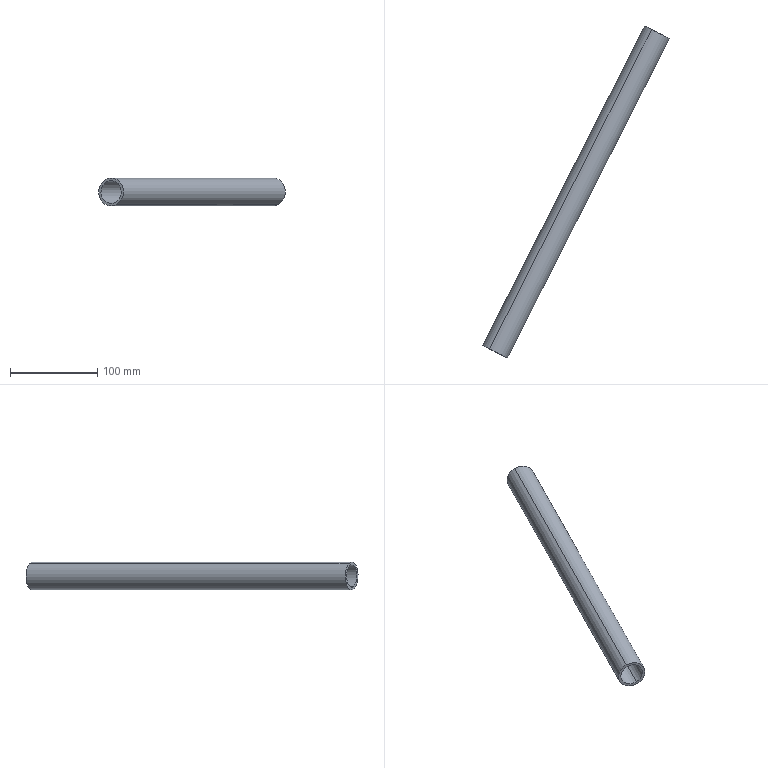Component | SolidWorks | WeldedPipe-1 | 1 solid | 6 faces | box 213.9 x 380.17 x 32 mm | volume 112061 mm3 | cylinder 4 | plane 2 | commonest cylinder face diameters 26 x2 32 x2
build123d program:
from build123d import *

# Parameters (mm, degrees)
SKETCH1_R           = 16
SKETCH1_R_2         = 13
BOSS_EXTRUDE1_DEPTH = 410


with BuildPart() as part:
    # Sketch1 → Boss-Extrude1 (new body)
    with BuildSketch(Plane(origin=(0, 0, 0), x_dir=(1, 0, 0), z_dir=(0, 1, 0))):
        with Locations(Location((0, 0, 0), (0, 0, 90))):
            Circle(SKETCH1_R)
        with Locations(Location((0, 0, 0), (0, 0, 90))):
            Circle(SKETCH1_R_2, mode=Mode.SUBTRACT)
    extrude(amount=BOSS_EXTRUDE1_DEPTH)


solid = part.part

# Placed as in the assembly
solid = solid.moved(Location((366.069, -1101.171, 1812.971), (12.669, 23.398, -29.512)))
STEP:
#1=COLOUR_RGB('',0.7922,0.8196,0.9333);
#2=FILL_AREA_STYLE_COLOUR('',#1);
#3=FILL_AREA_STYLE('',(#2));
#4=SURFACE_STYLE_FILL_AREA(#3);
#5=SURFACE_SIDE_STYLE('',(#4));
#6=SURFACE_STYLE_USAGE(.BOTH.,#5);
#7=PRESENTATION_STYLE_ASSIGNMENT((#6));
#8=CARTESIAN_POINT('',(21.904,-29.054,70.914));
#9=VERTEX_POINT('',#8);
#10=CARTESIAN_POINT('',(21.516,-28.857,71.84));
#11=VERTEX_POINT('',#10);
#12=CARTESIAN_POINT('',(21.71,-28.955,71.377));
#13=DIRECTION('',(0.4521,0.892,0.));
#14=DIRECTION('',(-0.3796,0.1924,0.9049));
#15=AXIS2_PLACEMENT_3D('',#12,#13,#14);
#16=CIRCLE('',#15,0.5118);
#17=EDGE_CURVE('',#9,#11,#16,.T.);
#18=ORIENTED_EDGE('',*,*,#17,.T.);
#19=CARTESIAN_POINT('',(14.218,-43.255,71.84));
#20=VERTEX_POINT('',#19);
#21=CARTESIAN_POINT('',(21.516,-28.857,71.84));
#22=DIRECTION('',(-0.4521,-0.892,-0.));
#23=VECTOR('',#22,39.37);
#24=LINE('',#21,#23);
#25=EDGE_CURVE('',#11,#20,#24,.T.);
#26=ORIENTED_EDGE('',*,*,#25,.T.);
#27=CARTESIAN_POINT('',(14.606,-43.452,70.914));
#28=VERTEX_POINT('',#27);
#29=CARTESIAN_POINT('',(14.412,-43.353,71.377));
#30=DIRECTION('',(0.4521,0.892,0.));
#31=DIRECTION('',(-0.3796,0.1924,0.9049));
#32=AXIS2_PLACEMENT_3D('',#29,#30,#31);
#33=CIRCLE('',#32,0.5118);
#34=EDGE_CURVE('',#28,#20,#33,.T.);
#35=ORIENTED_EDGE('',*,*,#34,.F.);
#36=CARTESIAN_POINT('',(21.904,-29.054,70.914));
#37=DIRECTION('',(-0.4521,-0.892,-0.));
#38=VECTOR('',#37,39.37);
#39=LINE('',#36,#38);
#40=EDGE_CURVE('',#9,#28,#39,.T.);
#41=ORIENTED_EDGE('',*,*,#40,.F.);
#42=EDGE_LOOP('',(#18,#26,#35,#41));
#43=FACE_OUTER_BOUND('',#42,.T.);
#44=CARTESIAN_POINT('',(21.71,-28.955,71.377));
#45=DIRECTION('',(-0.4521,-0.892,-0.));
#46=DIRECTION('',(0.3796,-0.1924,-0.9049));
#47=AXIS2_PLACEMENT_3D('',#44,#45,#46);
#48=CYLINDRICAL_SURFACE('',#47,0.5118);
#49=ADVANCED_FACE('',(#43),#48,.F.);
#50=CARTESIAN_POINT('',(21.471,-28.834,71.947));
#51=VERTEX_POINT('',#50);
#52=CARTESIAN_POINT('',(21.949,-29.077,70.807));
#53=VERTEX_POINT('',#52);
#54=CARTESIAN_POINT('',(21.71,-28.955,71.377));
#55=DIRECTION('',(0.4521,0.892,0.));
#56=DIRECTION('',(-0.3796,0.1924,0.9049));
#57=AXIS2_PLACEMENT_3D('',#54,#55,#56);
#58=CIRCLE('',#57,0.6299);
#59=EDGE_CURVE('',#51,#53,#58,.T.);
#60=ORIENTED_EDGE('',*,*,#59,.F.);
#61=CARTESIAN_POINT('',(14.173,-43.232,71.947));
#62=VERTEX_POINT('',#61);
#63=CARTESIAN_POINT('',(21.471,-28.834,71.947));
#64=DIRECTION('',(-0.4521,-0.892,-0.));
#65=VECTOR('',#64,39.37);
#66=LINE('',#63,#65);
#67=EDGE_CURVE('',#51,#62,#66,.T.);
#68=ORIENTED_EDGE('',*,*,#67,.T.);
#69=CARTESIAN_POINT('',(14.651,-43.474,70.807));
#70=VERTEX_POINT('',#69);
#71=CARTESIAN_POINT('',(14.412,-43.353,71.377));
#72=DIRECTION('',(0.4521,0.892,0.));
#73=DIRECTION('',(-0.3796,0.1924,0.9049));
#74=AXIS2_PLACEMENT_3D('',#71,#72,#73);
#75=CIRCLE('',#74,0.6299);
#76=EDGE_CURVE('',#62,#70,#75,.T.);
#77=ORIENTED_EDGE('',*,*,#76,.T.);
#78=CARTESIAN_POINT('',(21.949,-29.077,70.807));
#79=DIRECTION('',(-0.4521,-0.892,-0.));
#80=VECTOR('',#79,39.37);
#81=LINE('',#78,#80);
#82=EDGE_CURVE('',#53,#70,#81,.T.);
#83=ORIENTED_EDGE('',*,*,#82,.F.);
#84=EDGE_LOOP('',(#60,#68,#77,#83));
#85=FACE_OUTER_BOUND('',#84,.T.);
#86=CARTESIAN_POINT('',(21.71,-28.955,71.377));
#87=DIRECTION('',(-0.4521,-0.892,-0.));
#88=DIRECTION('',(0.3796,-0.1924,-0.9049));
#89=AXIS2_PLACEMENT_3D('',#86,#87,#88);
#90=CYLINDRICAL_SURFACE('',#89,0.6299);
#91=ADVANCED_FACE('',(#85),#90,.T.);
#92=CARTESIAN_POINT('',(21.71,-28.955,71.377));
#93=DIRECTION('',(0.4521,0.892,0.));
#94=DIRECTION('',(-0.3796,0.1924,0.9049));
#95=AXIS2_PLACEMENT_3D('',#92,#93,#94);
#96=CIRCLE('',#95,0.6299);
#97=EDGE_CURVE('',#53,#51,#96,.T.);
#98=ORIENTED_EDGE('',*,*,#97,.T.);
#99=ORIENTED_EDGE('',*,*,#59,.T.);
#100=EDGE_LOOP('',(#98,#99));
#101=FACE_OUTER_BOUND('',#100,.T.);
#102=ORIENTED_EDGE('',*,*,#17,.F.);
#103=CARTESIAN_POINT('',(21.71,-28.955,71.377));
#104=DIRECTION('',(0.4521,0.892,0.));
#105=DIRECTION('',(-0.3796,0.1924,0.9049));
#106=AXIS2_PLACEMENT_3D('',#103,#104,#105);
#107=CIRCLE('',#106,0.5118);
#108=EDGE_CURVE('',#11,#9,#107,.T.);
#109=ORIENTED_EDGE('',*,*,#108,.F.);
#110=EDGE_LOOP('',(#102,#109));
#111=FACE_BOUND('',#110,.T.);
#112=CARTESIAN_POINT('',(21.71,-28.955,71.377));
#113=DIRECTION('',(0.4521,0.892,0.));
#114=DIRECTION('',(-0.3796,0.1924,0.9049));
#115=AXIS2_PLACEMENT_3D('',#112,#113,#114);
#116=PLANE('',#115);
#117=ADVANCED_FACE('',(#101,#111),#116,.T.);
#118=CARTESIAN_POINT('',(14.412,-43.353,71.377));
#119=DIRECTION('',(0.4521,0.892,0.));
#120=DIRECTION('',(-0.3796,0.1924,0.9049));
#121=AXIS2_PLACEMENT_3D('',#118,#119,#120);
#122=CIRCLE('',#121,0.6299);
#123=EDGE_CURVE('',#70,#62,#122,.T.);
#124=ORIENTED_EDGE('',*,*,#123,.F.);
#125=ORIENTED_EDGE('',*,*,#76,.F.);
#126=EDGE_LOOP('',(#124,#125));
#127=FACE_OUTER_BOUND('',#126,.T.);
#128=ORIENTED_EDGE('',*,*,#34,.T.);
#129=CARTESIAN_POINT('',(14.412,-43.353,71.377));
#130=DIRECTION('',(0.4521,0.892,0.));
#131=DIRECTION('',(-0.3796,0.1924,0.9049));
#132=AXIS2_PLACEMENT_3D('',#129,#130,#131);
#133=CIRCLE('',#132,0.5118);
#134=EDGE_CURVE('',#20,#28,#133,.T.);
#135=ORIENTED_EDGE('',*,*,#134,.T.);
#136=EDGE_LOOP('',(#128,#135));
#137=FACE_BOUND('',#136,.T.);
#138=CARTESIAN_POINT('',(14.412,-43.353,71.377));
#139=DIRECTION('',(0.4521,0.892,0.));
#140=DIRECTION('',(-0.3796,0.1924,0.9049));
#141=AXIS2_PLACEMENT_3D('',#138,#139,#140);
#142=PLANE('',#141);
#143=ADVANCED_FACE('',(#127,#137),#142,.F.);
#144=ORIENTED_EDGE('',*,*,#67,.F.);
#145=ORIENTED_EDGE('',*,*,#97,.F.);
#146=ORIENTED_EDGE('',*,*,#82,.T.);
#147=ORIENTED_EDGE('',*,*,#123,.T.);
#148=EDGE_LOOP('',(#144,#145,#146,#147));
#149=FACE_OUTER_BOUND('',#148,.T.);
#150=CARTESIAN_POINT('',(21.71,-28.955,71.377));
#151=DIRECTION('',(-0.4521,-0.892,-0.));
#152=DIRECTION('',(0.3796,-0.1924,-0.9049));
#153=AXIS2_PLACEMENT_3D('',#150,#151,#152);
#154=CYLINDRICAL_SURFACE('',#153,0.6299);
#155=ADVANCED_FACE('',(#149),#154,.T.);
#156=ORIENTED_EDGE('',*,*,#25,.F.);
#157=ORIENTED_EDGE('',*,*,#108,.T.);
#158=ORIENTED_EDGE('',*,*,#40,.T.);
#159=ORIENTED_EDGE('',*,*,#134,.F.);
#160=EDGE_LOOP('',(#156,#157,#158,#159));
#161=FACE_OUTER_BOUND('',#160,.T.);
#162=CARTESIAN_POINT('',(21.71,-28.955,71.377));
#163=DIRECTION('',(-0.4521,-0.892,-0.));
#164=DIRECTION('',(0.3796,-0.1924,-0.9049));
#165=AXIS2_PLACEMENT_3D('',#162,#163,#164);
#166=CYLINDRICAL_SURFACE('',#165,0.5118);
#167=ADVANCED_FACE('',(#161),#166,.F.);
#168=CLOSED_SHELL('',(#49,#91,#117,#143,#155,#167));
#169=MANIFOLD_SOLID_BREP('',#168);
#170=STYLED_ITEM('',(#7),#169);
#171=(LENGTH_UNIT()NAMED_UNIT(*)SI_UNIT($,.METRE.));
#172=LENGTH_MEASURE_WITH_UNIT(LENGTH_MEASURE(0.0254),#171);
#173=DIMENSIONAL_EXPONENTS(1.,0.,0.,0.,0.,0.,0.);
#174=(CONVERSION_BASED_UNIT('',#172)LENGTH_UNIT()NAMED_UNIT(#173));
#175=UNCERTAINTY_MEASURE_WITH_UNIT(LENGTH_MEASURE(0.00001),#174,'','');
#176=(NAMED_UNIT(*)PLANE_ANGLE_UNIT()SI_UNIT($,.RADIAN.));
#177=(NAMED_UNIT(*)SI_UNIT($,.STERADIAN.)SOLID_ANGLE_UNIT());
#178=(GEOMETRIC_REPRESENTATION_CONTEXT(3)GLOBAL_UNCERTAINTY_ASSIGNED_CONTEXT((#175))GLOBAL_UNIT_ASSIGNED_CONTEXT((#174,#176,#177))REPRESENTATION_CONTEXT('',''));
#179=MECHANICAL_DESIGN_GEOMETRIC_PRESENTATION_REPRESENTATION('',(#170),#178);
#180=CARTESIAN_POINT('',(0.,0.,0.));
#181=DIRECTION('',(0.,0.,1.));
#182=DIRECTION('',(1.,0.,0.));
#183=AXIS2_PLACEMENT_3D('',#180,#181,#182);
#184=(LENGTH_UNIT()NAMED_UNIT(*)SI_UNIT($,.METRE.));
#185=LENGTH_MEASURE_WITH_UNIT(LENGTH_MEASURE(0.0254),#184);
#186=DIMENSIONAL_EXPONENTS(1.,0.,0.,0.,0.,0.,0.);
#187=(CONVERSION_BASED_UNIT('',#185)LENGTH_UNIT()NAMED_UNIT(#186));
#188=UNCERTAINTY_MEASURE_WITH_UNIT(LENGTH_MEASURE(0.00001),#187,'','');
#189=(NAMED_UNIT(*)PLANE_ANGLE_UNIT()SI_UNIT($,.RADIAN.));
#190=(NAMED_UNIT(*)SI_UNIT($,.STERADIAN.)SOLID_ANGLE_UNIT());
#191=(GEOMETRIC_REPRESENTATION_CONTEXT(3)GLOBAL_UNCERTAINTY_ASSIGNED_CONTEXT((#188))GLOBAL_UNIT_ASSIGNED_CONTEXT((#187,#189,#190))REPRESENTATION_CONTEXT('',''));
#192=ADVANCED_BREP_SHAPE_REPRESENTATION('',(#169,#183),#191);
#193=PRESENTATION_LAYER_ASSIGNMENT('','',(#170));